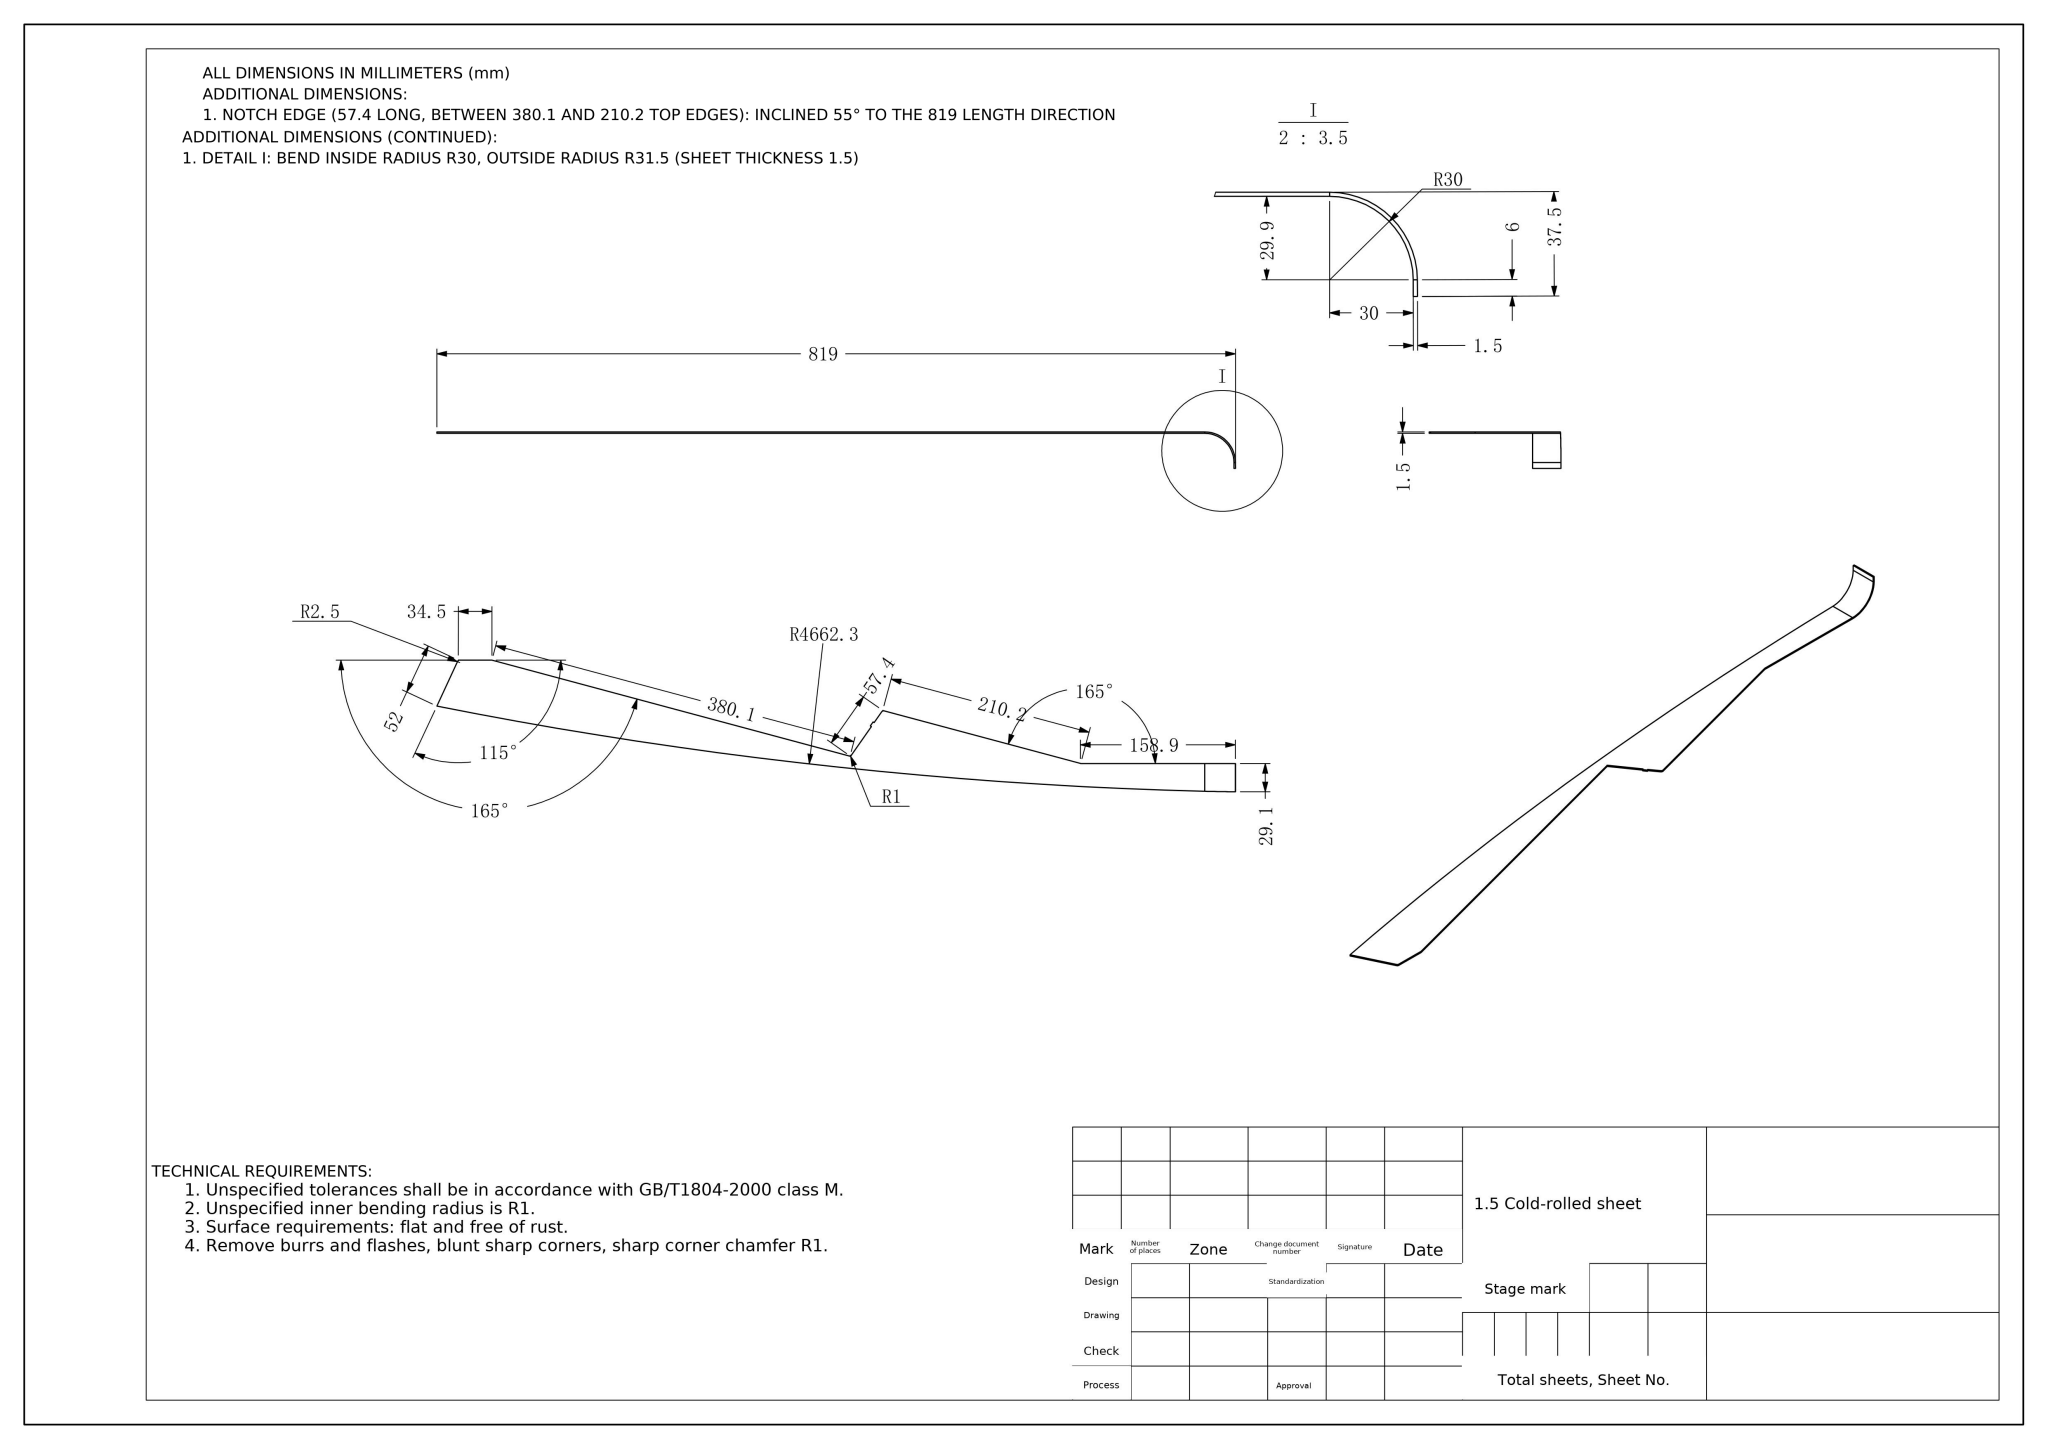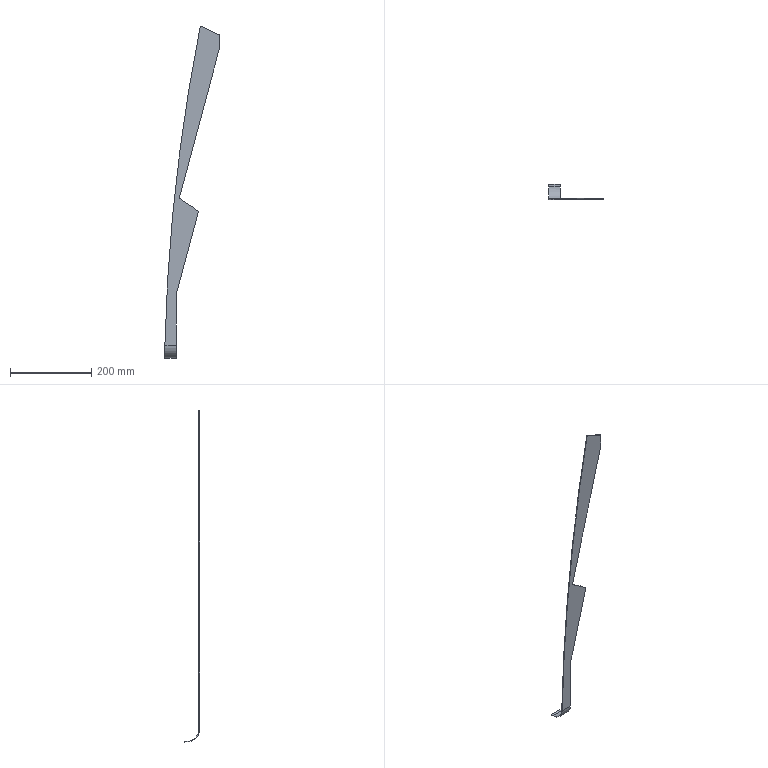Part | NX | mm | 1 solid | 25 faces | box 135.07 x 37.4 x 818.96 mm | volume 47035 mm3 | plane 16 | cylinder 8 | spline 1 | commonest cylinder face diameters 5 x3 2 x2 9324.641 x1 63 x1 60 x1